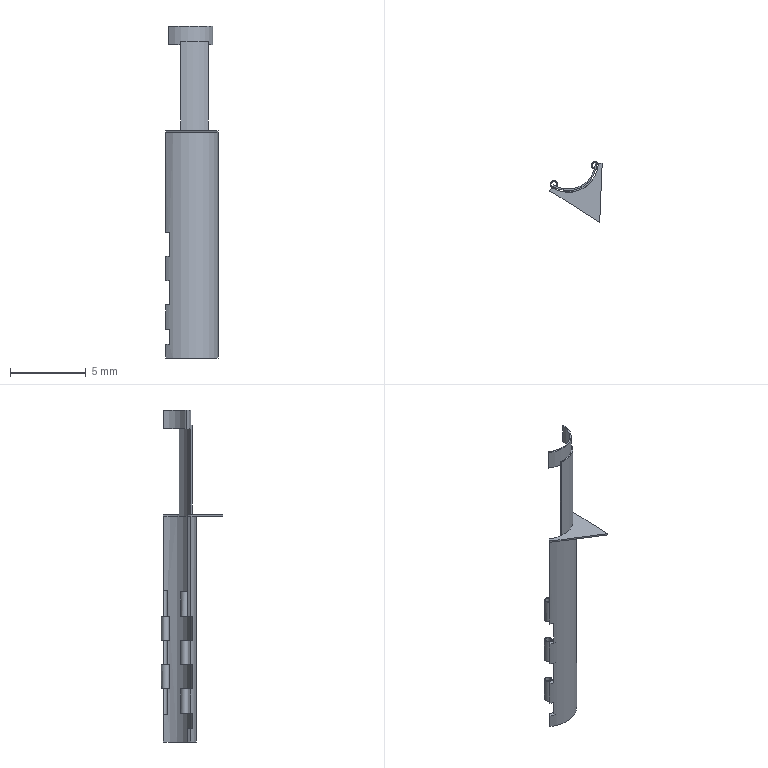Component | NX | MIDDLE_PART | 9 solids | 60 faces | volume 19 mm3 | plane 39 | cylinder 21 | commonest cylinder face diameters 0.5 x6 0.4 x5 4 x3 1.1 x3 3.8 x2 3.6 x1 4.5 x1